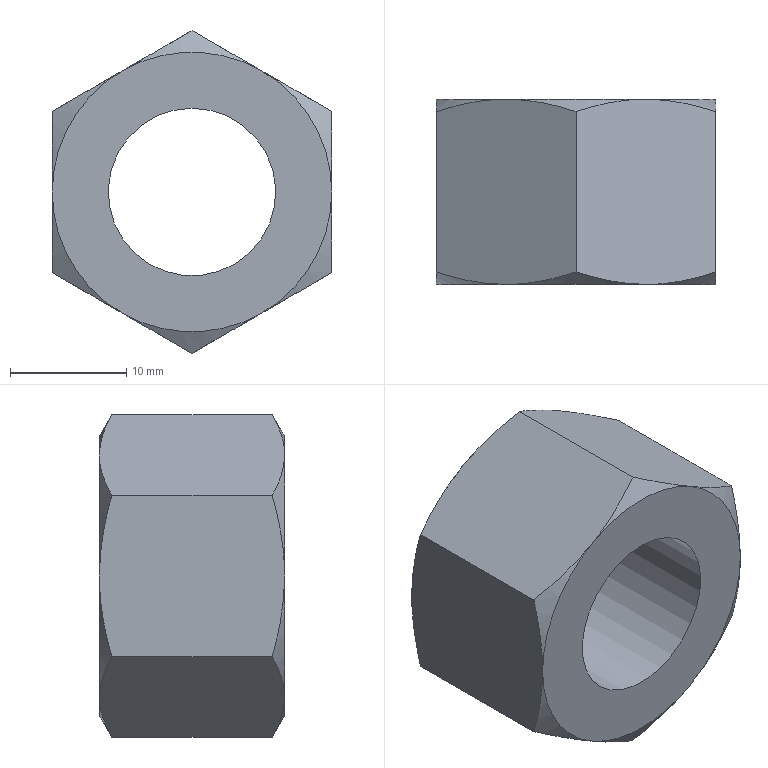Component | NX | GB-T41-2000_M16X2 | 1 solid | 21 faces | volume 5320 mm3 | cone 12 | plane 8 | cylinder 1 | commonest cylinder face diameters 14.376 x1